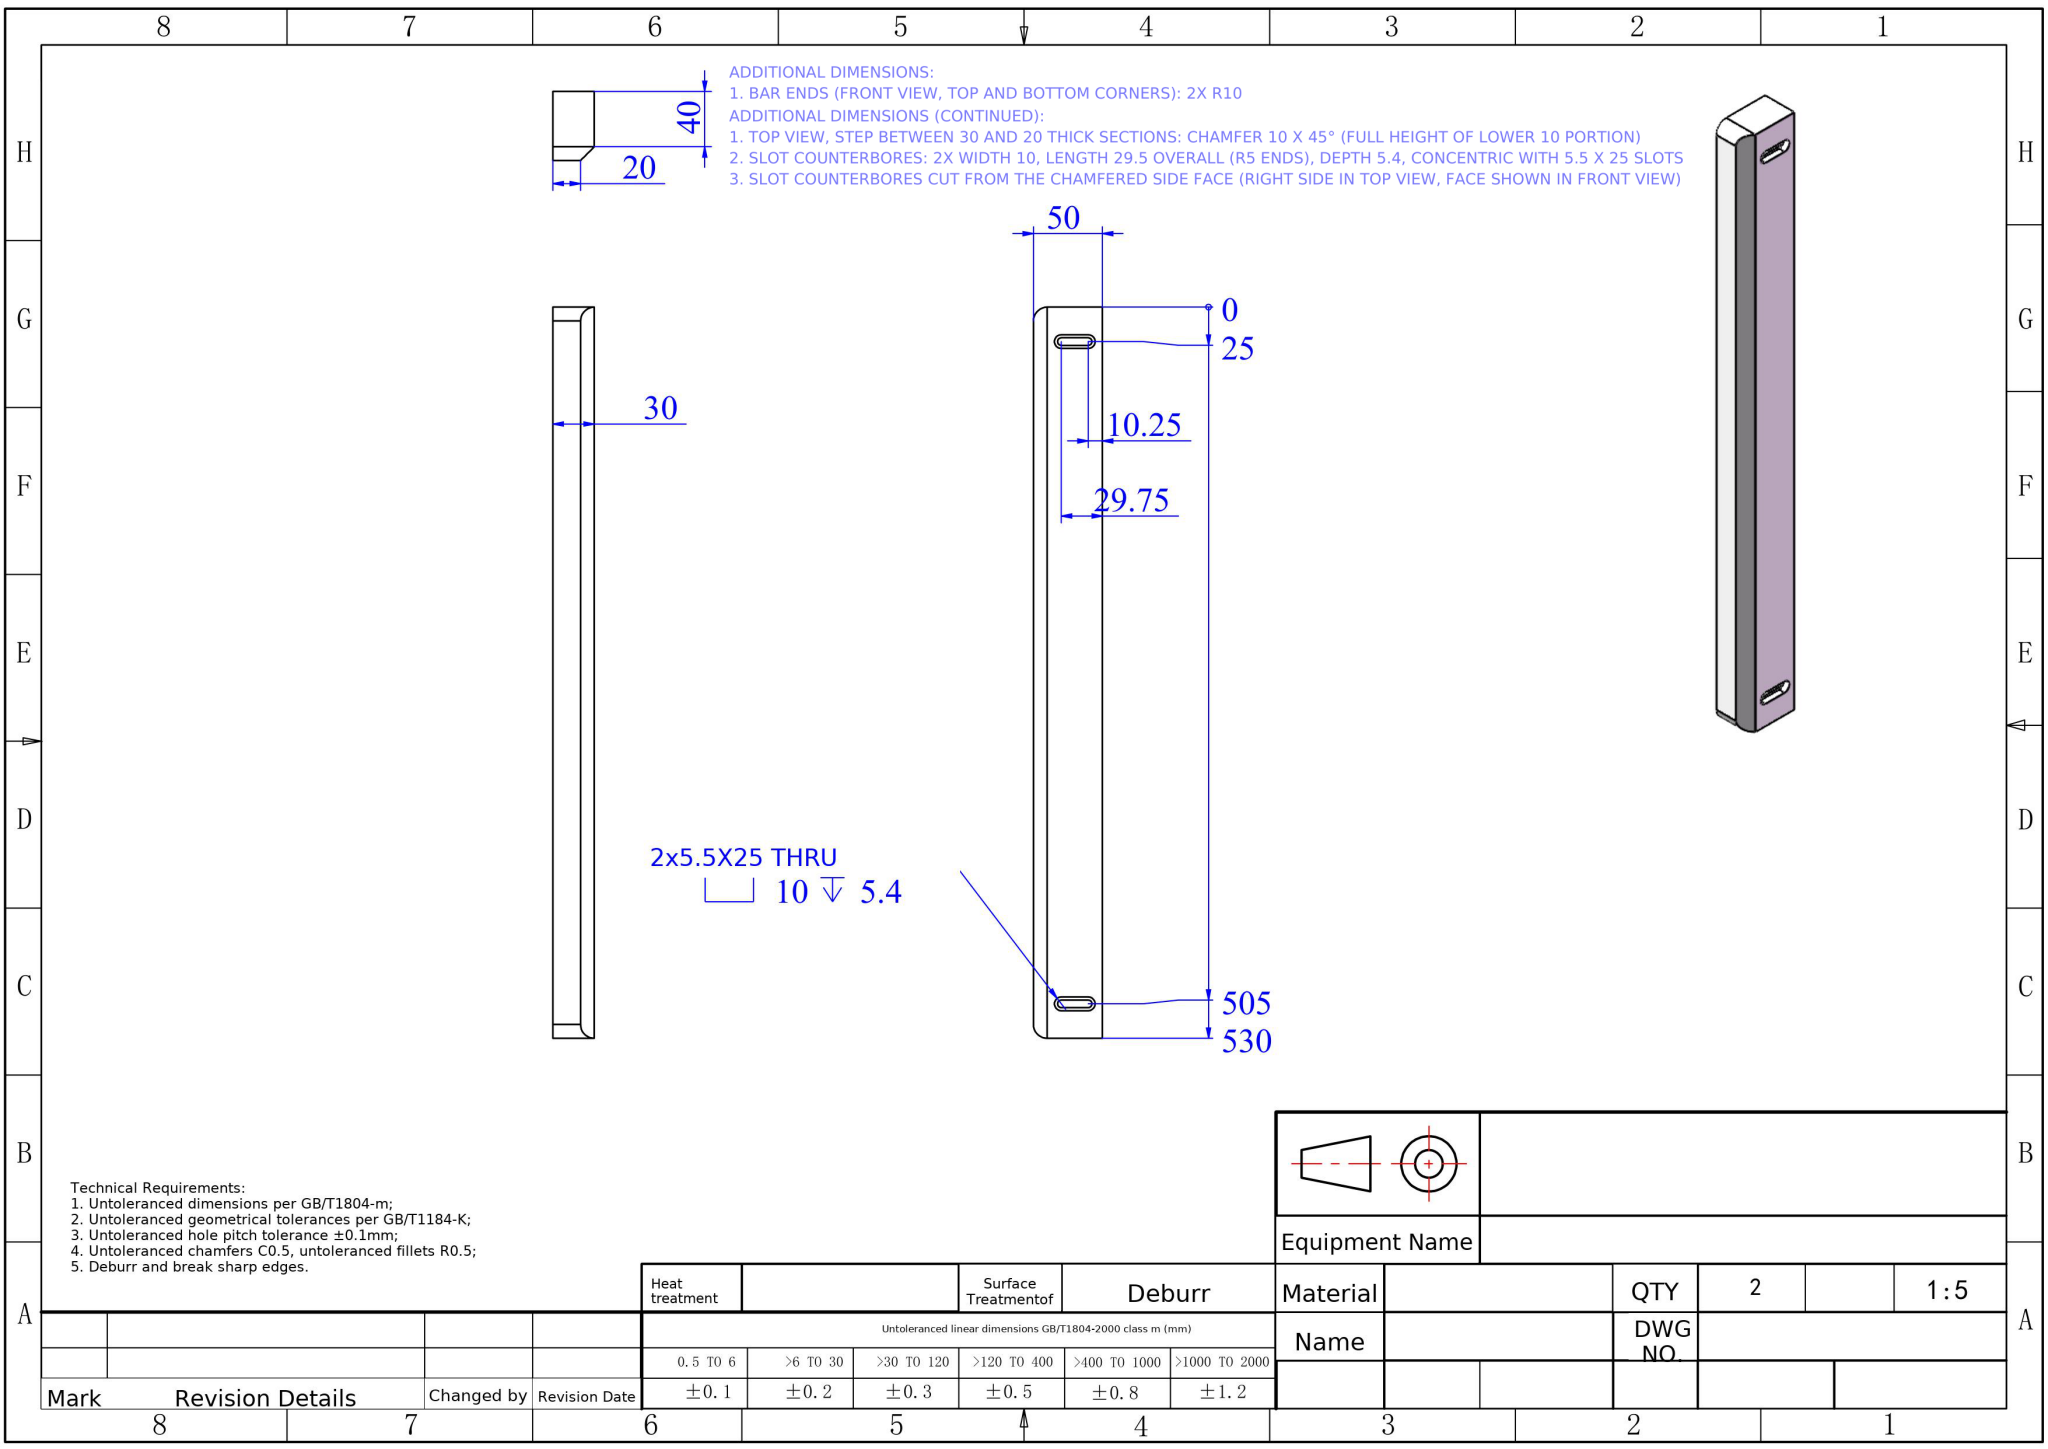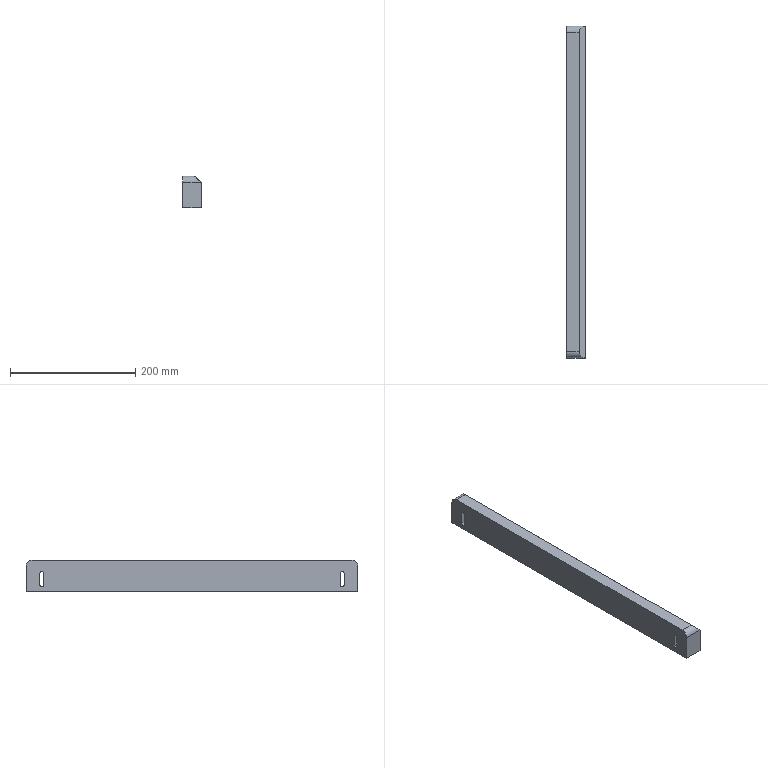Part | NX | mm | 1 solid | 31 faces | box 30 x 530 x 50 mm | volume 758146 mm3 | plane 17 | cylinder 14 | commonest cylinder face diameters 10 x6 5.5 x6 20 x2
STEP:
#1=CARTESIAN_POINT('',(9.6,-240.,5.25));
#2=VERTEX_POINT('',#1);
#3=CARTESIAN_POINT('',(9.6,-235.,10.25));
#4=VERTEX_POINT('',#3);
#5=CARTESIAN_POINT('',(9.6,-240.,10.25));
#6=DIRECTION('',(1.,0.,0.));
#7=DIRECTION('',(0.,0.,-1.));
#8=AXIS2_PLACEMENT_3D('',#5,#6,#7);
#9=CIRCLE('',#8,5.);
#10=EDGE_CURVE('',#2,#4,#9,.T.);
#11=ORIENTED_EDGE('',*,*,#10,.F.);
#12=CARTESIAN_POINT('',(15.,-240.,5.25));
#13=VERTEX_POINT('',#12);
#14=CARTESIAN_POINT('',(15.,-240.,5.25));
#15=DIRECTION('',(1.,0.,0.));
#16=VECTOR('',#15,1000.);
#17=LINE('',#14,#16);
#18=EDGE_CURVE('',#2,#13,#17,.T.);
#19=ORIENTED_EDGE('',*,*,#18,.T.);
#20=CARTESIAN_POINT('',(15.,-235.,10.25));
#21=VERTEX_POINT('',#20);
#22=CARTESIAN_POINT('',(15.,-240.,10.25));
#23=DIRECTION('',(1.,0.,0.));
#24=DIRECTION('',(0.,0.,-1.));
#25=AXIS2_PLACEMENT_3D('',#22,#23,#24);
#26=CIRCLE('',#25,5.);
#27=EDGE_CURVE('',#13,#21,#26,.T.);
#28=ORIENTED_EDGE('',*,*,#27,.T.);
#29=CARTESIAN_POINT('',(9.6,-235.,10.25));
#30=DIRECTION('',(-1.,-0.,0.));
#31=VECTOR('',#30,1000.);
#32=LINE('',#29,#31);
#33=EDGE_CURVE('',#21,#4,#32,.T.);
#34=ORIENTED_EDGE('',*,*,#33,.T.);
#35=EDGE_LOOP('',(#11,#19,#28,#34));
#36=FACE_OUTER_BOUND('',#35,.T.);
#37=CARTESIAN_POINT('',(15.,-240.,10.25));
#38=DIRECTION('',(1.,0.,0.));
#39=DIRECTION('',(0.,0.,-1.));
#40=AXIS2_PLACEMENT_3D('',#37,#38,#39);
#41=CYLINDRICAL_SURFACE('',#40,5.);
#42=ADVANCED_FACE('',(#36),#41,.F.);
#43=CARTESIAN_POINT('',(-15.,-240.,7.5));
#44=VERTEX_POINT('',#43);
#45=CARTESIAN_POINT('',(-15.,-237.25,10.25));
#46=VERTEX_POINT('',#45);
#47=CARTESIAN_POINT('',(-15.,-240.,10.25));
#48=DIRECTION('',(1.,0.,0.));
#49=DIRECTION('',(0.,0.,-1.));
#50=AXIS2_PLACEMENT_3D('',#47,#48,#49);
#51=CIRCLE('',#50,2.75);
#52=EDGE_CURVE('',#44,#46,#51,.T.);
#53=ORIENTED_EDGE('',*,*,#52,.F.);
#54=CARTESIAN_POINT('',(9.6,-240.,7.5));
#55=VERTEX_POINT('',#54);
#56=CARTESIAN_POINT('',(15.,-240.,7.5));
#57=DIRECTION('',(1.,0.,0.));
#58=VECTOR('',#57,1000.);
#59=LINE('',#56,#58);
#60=EDGE_CURVE('',#44,#55,#59,.T.);
#61=ORIENTED_EDGE('',*,*,#60,.T.);
#62=CARTESIAN_POINT('',(9.6,-237.25,10.25));
#63=VERTEX_POINT('',#62);
#64=CARTESIAN_POINT('',(9.6,-240.,10.25));
#65=DIRECTION('',(1.,0.,0.));
#66=DIRECTION('',(0.,0.,-1.));
#67=AXIS2_PLACEMENT_3D('',#64,#65,#66);
#68=CIRCLE('',#67,2.75);
#69=EDGE_CURVE('',#55,#63,#68,.T.);
#70=ORIENTED_EDGE('',*,*,#69,.T.);
#71=CARTESIAN_POINT('',(-15.,-237.25,10.25));
#72=DIRECTION('',(-1.,-0.,0.));
#73=VECTOR('',#72,1000.);
#74=LINE('',#71,#73);
#75=EDGE_CURVE('',#63,#46,#74,.T.);
#76=ORIENTED_EDGE('',*,*,#75,.T.);
#77=EDGE_LOOP('',(#53,#61,#70,#76));
#78=FACE_OUTER_BOUND('',#77,.T.);
#79=CARTESIAN_POINT('',(15.,-240.,10.25));
#80=DIRECTION('',(1.,0.,0.));
#81=DIRECTION('',(0.,0.,-1.));
#82=AXIS2_PLACEMENT_3D('',#79,#80,#81);
#83=CYLINDRICAL_SURFACE('',#82,2.75);
#84=ADVANCED_FACE('',(#78),#83,.F.);
#85=CARTESIAN_POINT('',(9.6,240.,5.25));
#86=VERTEX_POINT('',#85);
#87=CARTESIAN_POINT('',(9.6,245.,10.25));
#88=VERTEX_POINT('',#87);
#89=CARTESIAN_POINT('',(9.6,240.,10.25));
#90=DIRECTION('',(1.,0.,0.));
#91=DIRECTION('',(0.,0.,-1.));
#92=AXIS2_PLACEMENT_3D('',#89,#90,#91);
#93=CIRCLE('',#92,5.);
#94=EDGE_CURVE('',#86,#88,#93,.T.);
#95=ORIENTED_EDGE('',*,*,#94,.F.);
#96=CARTESIAN_POINT('',(15.,240.,5.25));
#97=VERTEX_POINT('',#96);
#98=CARTESIAN_POINT('',(15.,240.,5.25));
#99=DIRECTION('',(1.,0.,0.));
#100=VECTOR('',#99,1000.);
#101=LINE('',#98,#100);
#102=EDGE_CURVE('',#86,#97,#101,.T.);
#103=ORIENTED_EDGE('',*,*,#102,.T.);
#104=CARTESIAN_POINT('',(15.,245.,10.25));
#105=VERTEX_POINT('',#104);
#106=CARTESIAN_POINT('',(15.,240.,10.25));
#107=DIRECTION('',(1.,0.,0.));
#108=DIRECTION('',(0.,0.,-1.));
#109=AXIS2_PLACEMENT_3D('',#106,#107,#108);
#110=CIRCLE('',#109,5.);
#111=EDGE_CURVE('',#97,#105,#110,.T.);
#112=ORIENTED_EDGE('',*,*,#111,.T.);
#113=CARTESIAN_POINT('',(9.6,245.,10.25));
#114=DIRECTION('',(-1.,-0.,0.));
#115=VECTOR('',#114,1000.);
#116=LINE('',#113,#115);
#117=EDGE_CURVE('',#105,#88,#116,.T.);
#118=ORIENTED_EDGE('',*,*,#117,.T.);
#119=EDGE_LOOP('',(#95,#103,#112,#118));
#120=FACE_OUTER_BOUND('',#119,.T.);
#121=CARTESIAN_POINT('',(15.,240.,10.25));
#122=DIRECTION('',(1.,0.,0.));
#123=DIRECTION('',(0.,0.,-1.));
#124=AXIS2_PLACEMENT_3D('',#121,#122,#123);
#125=CYLINDRICAL_SURFACE('',#124,5.);
#126=ADVANCED_FACE('',(#120),#125,.F.);
#127=CARTESIAN_POINT('',(-15.,240.,7.5));
#128=VERTEX_POINT('',#127);
#129=CARTESIAN_POINT('',(-15.,242.75,10.25));
#130=VERTEX_POINT('',#129);
#131=CARTESIAN_POINT('',(-15.,240.,10.25));
#132=DIRECTION('',(1.,0.,0.));
#133=DIRECTION('',(0.,0.,-1.));
#134=AXIS2_PLACEMENT_3D('',#131,#132,#133);
#135=CIRCLE('',#134,2.75);
#136=EDGE_CURVE('',#128,#130,#135,.T.);
#137=ORIENTED_EDGE('',*,*,#136,.F.);
#138=CARTESIAN_POINT('',(9.6,240.,7.5));
#139=VERTEX_POINT('',#138);
#140=CARTESIAN_POINT('',(15.,240.,7.5));
#141=DIRECTION('',(1.,0.,0.));
#142=VECTOR('',#141,1000.);
#143=LINE('',#140,#142);
#144=EDGE_CURVE('',#128,#139,#143,.T.);
#145=ORIENTED_EDGE('',*,*,#144,.T.);
#146=CARTESIAN_POINT('',(9.6,242.75,10.25));
#147=VERTEX_POINT('',#146);
#148=CARTESIAN_POINT('',(9.6,240.,10.25));
#149=DIRECTION('',(1.,0.,0.));
#150=DIRECTION('',(0.,0.,-1.));
#151=AXIS2_PLACEMENT_3D('',#148,#149,#150);
#152=CIRCLE('',#151,2.75);
#153=EDGE_CURVE('',#139,#147,#152,.T.);
#154=ORIENTED_EDGE('',*,*,#153,.T.);
#155=CARTESIAN_POINT('',(-15.,242.75,10.25));
#156=DIRECTION('',(-1.,-0.,0.));
#157=VECTOR('',#156,1000.);
#158=LINE('',#155,#157);
#159=EDGE_CURVE('',#147,#130,#158,.T.);
#160=ORIENTED_EDGE('',*,*,#159,.T.);
#161=EDGE_LOOP('',(#137,#145,#154,#160));
#162=FACE_OUTER_BOUND('',#161,.T.);
#163=CARTESIAN_POINT('',(15.,240.,10.25));
#164=DIRECTION('',(1.,0.,0.));
#165=DIRECTION('',(0.,0.,-1.));
#166=AXIS2_PLACEMENT_3D('',#163,#164,#165);
#167=CYLINDRICAL_SURFACE('',#166,2.75);
#168=ADVANCED_FACE('',(#162),#167,.F.);
#169=CARTESIAN_POINT('',(15.,-245.,10.25));
#170=VERTEX_POINT('',#169);
#171=CARTESIAN_POINT('',(15.,-240.,10.25));
#172=DIRECTION('',(1.,0.,0.));
#173=DIRECTION('',(0.,0.,-1.));
#174=AXIS2_PLACEMENT_3D('',#171,#172,#173);
#175=CIRCLE('',#174,5.);
#176=EDGE_CURVE('',#170,#13,#175,.T.);
#177=ORIENTED_EDGE('',*,*,#176,.F.);
#178=CARTESIAN_POINT('',(15.,-245.,29.75));
#179=VERTEX_POINT('',#178);
#180=CARTESIAN_POINT('',(15.,-245.,10.25));
#181=DIRECTION('',(0.,0.,1.));
#182=VECTOR('',#181,1000.);
#183=LINE('',#180,#182);
#184=EDGE_CURVE('',#170,#179,#183,.T.);
#185=ORIENTED_EDGE('',*,*,#184,.T.);
#186=CARTESIAN_POINT('',(15.,-235.,29.75));
#187=VERTEX_POINT('',#186);
#188=CARTESIAN_POINT('',(15.,-240.,29.75));
#189=DIRECTION('',(1.,0.,0.));
#190=DIRECTION('',(0.,0.,-1.));
#191=AXIS2_PLACEMENT_3D('',#188,#189,#190);
#192=CIRCLE('',#191,5.);
#193=EDGE_CURVE('',#187,#179,#192,.T.);
#194=ORIENTED_EDGE('',*,*,#193,.F.);
#195=CARTESIAN_POINT('',(15.,-235.,10.25));
#196=DIRECTION('',(0.,0.,1.));
#197=VECTOR('',#196,1000.);
#198=LINE('',#195,#197);
#199=EDGE_CURVE('',#21,#187,#198,.T.);
#200=ORIENTED_EDGE('',*,*,#199,.F.);
#201=ORIENTED_EDGE('',*,*,#27,.F.);
#202=EDGE_LOOP('',(#177,#185,#194,#200,#201));
#203=FACE_BOUND('',#202,.T.);
#204=CARTESIAN_POINT('',(15.,265.,40.));
#205=VERTEX_POINT('',#204);
#206=CARTESIAN_POINT('',(15.,265.,0.));
#207=VERTEX_POINT('',#206);
#208=CARTESIAN_POINT('',(15.,265.,50.));
#209=DIRECTION('',(0.,0.,-1.));
#210=VECTOR('',#209,1000.);
#211=LINE('',#208,#210);
#212=EDGE_CURVE('',#205,#207,#211,.T.);
#213=ORIENTED_EDGE('',*,*,#212,.F.);
#214=CARTESIAN_POINT('',(15.,-265.,40.));
#215=VERTEX_POINT('',#214);
#216=CARTESIAN_POINT('',(15.,-265.,40.));
#217=DIRECTION('',(0.,-1.,0.));
#218=VECTOR('',#217,1000.);
#219=LINE('',#216,#218);
#220=EDGE_CURVE('',#205,#215,#219,.T.);
#221=ORIENTED_EDGE('',*,*,#220,.T.);
#222=CARTESIAN_POINT('',(15.,-265.,0.));
#223=VERTEX_POINT('',#222);
#224=CARTESIAN_POINT('',(15.,-265.,50.));
#225=DIRECTION('',(0.,0.,-1.));
#226=VECTOR('',#225,1000.);
#227=LINE('',#224,#226);
#228=EDGE_CURVE('',#215,#223,#227,.T.);
#229=ORIENTED_EDGE('',*,*,#228,.T.);
#230=CARTESIAN_POINT('',(15.,-265.,0.));
#231=DIRECTION('',(0.,1.,0.));
#232=VECTOR('',#231,1000.);
#233=LINE('',#230,#232);
#234=EDGE_CURVE('',#223,#207,#233,.T.);
#235=ORIENTED_EDGE('',*,*,#234,.T.);
#236=EDGE_LOOP('',(#213,#221,#229,#235));
#237=FACE_OUTER_BOUND('',#236,.T.);
#238=CARTESIAN_POINT('',(15.,245.,29.75));
#239=VERTEX_POINT('',#238);
#240=CARTESIAN_POINT('',(15.,245.,10.25));
#241=DIRECTION('',(0.,0.,1.));
#242=VECTOR('',#241,1000.);
#243=LINE('',#240,#242);
#244=EDGE_CURVE('',#105,#239,#243,.T.);
#245=ORIENTED_EDGE('',*,*,#244,.F.);
#246=ORIENTED_EDGE('',*,*,#111,.F.);
#247=CARTESIAN_POINT('',(15.,235.,10.25));
#248=VERTEX_POINT('',#247);
#249=CARTESIAN_POINT('',(15.,240.,10.25));
#250=DIRECTION('',(1.,0.,0.));
#251=DIRECTION('',(0.,0.,-1.));
#252=AXIS2_PLACEMENT_3D('',#249,#250,#251);
#253=CIRCLE('',#252,5.);
#254=EDGE_CURVE('',#248,#97,#253,.T.);
#255=ORIENTED_EDGE('',*,*,#254,.F.);
#256=CARTESIAN_POINT('',(15.,235.,29.75));
#257=VERTEX_POINT('',#256);
#258=CARTESIAN_POINT('',(15.,235.,10.25));
#259=DIRECTION('',(0.,0.,1.));
#260=VECTOR('',#259,1000.);
#261=LINE('',#258,#260);
#262=EDGE_CURVE('',#248,#257,#261,.T.);
#263=ORIENTED_EDGE('',*,*,#262,.T.);
#264=CARTESIAN_POINT('',(15.,240.,29.75));
#265=DIRECTION('',(1.,0.,0.));
#266=DIRECTION('',(0.,0.,-1.));
#267=AXIS2_PLACEMENT_3D('',#264,#265,#266);
#268=CIRCLE('',#267,5.);
#269=EDGE_CURVE('',#239,#257,#268,.T.);
#270=ORIENTED_EDGE('',*,*,#269,.F.);
#271=EDGE_LOOP('',(#245,#246,#255,#263,#270));
#272=FACE_BOUND('',#271,.T.);
#273=CARTESIAN_POINT('',(15.,-265.,50.));
#274=DIRECTION('',(-1.,0.,0.));
#275=DIRECTION('',(0.,0.,1.));
#276=AXIS2_PLACEMENT_3D('',#273,#274,#275);
#277=PLANE('',#276);
#278=ADVANCED_FACE('',(#203,#237,#272),#277,.F.);
#279=CARTESIAN_POINT('',(-15.,265.,40.));
#280=VERTEX_POINT('',#279);
#281=CARTESIAN_POINT('',(-15.,265.,0.));
#282=VERTEX_POINT('',#281);
#283=CARTESIAN_POINT('',(-15.,265.,50.));
#284=DIRECTION('',(0.,0.,-1.));
#285=VECTOR('',#284,1000.);
#286=LINE('',#283,#285);
#287=EDGE_CURVE('',#280,#282,#286,.T.);
#288=ORIENTED_EDGE('',*,*,#287,.F.);
#289=CARTESIAN_POINT('',(-15.,265.,40.));
#290=DIRECTION('',(1.,0.,0.));
#291=VECTOR('',#290,1000.);
#292=LINE('',#289,#291);
#293=EDGE_CURVE('',#280,#205,#292,.T.);
#294=ORIENTED_EDGE('',*,*,#293,.T.);
#295=ORIENTED_EDGE('',*,*,#212,.T.);
#296=CARTESIAN_POINT('',(-15.,265.,0.));
#297=DIRECTION('',(-1.,0.,0.));
#298=VECTOR('',#297,1000.);
#299=LINE('',#296,#298);
#300=EDGE_CURVE('',#207,#282,#299,.T.);
#301=ORIENTED_EDGE('',*,*,#300,.T.);
#302=EDGE_LOOP('',(#288,#294,#295,#301));
#303=FACE_OUTER_BOUND('',#302,.T.);
#304=CARTESIAN_POINT('',(-15.,265.,50.));
#305=DIRECTION('',(0.,-1.,0.));
#306=DIRECTION('',(0.,0.,-1.));
#307=AXIS2_PLACEMENT_3D('',#304,#305,#306);
#308=PLANE('',#307);
#309=ADVANCED_FACE('',(#303),#308,.F.);
#310=CARTESIAN_POINT('',(-15.,-242.75,10.25));
#311=VERTEX_POINT('',#310);
#312=CARTESIAN_POINT('',(-15.,-242.75,29.75));
#313=VERTEX_POINT('',#312);
#314=CARTESIAN_POINT('',(-15.,-242.75,10.25));
#315=DIRECTION('',(0.,0.,1.));
#316=VECTOR('',#315,1000.);
#317=LINE('',#314,#316);
#318=EDGE_CURVE('',#311,#313,#317,.T.);
#319=ORIENTED_EDGE('',*,*,#318,.F.);
#320=CARTESIAN_POINT('',(-15.,-240.,10.25));
#321=DIRECTION('',(1.,0.,0.));
#322=DIRECTION('',(0.,0.,-1.));
#323=AXIS2_PLACEMENT_3D('',#320,#321,#322);
#324=CIRCLE('',#323,2.75);
#325=EDGE_CURVE('',#311,#44,#324,.T.);
#326=ORIENTED_EDGE('',*,*,#325,.T.);
#327=ORIENTED_EDGE('',*,*,#52,.T.);
#328=CARTESIAN_POINT('',(-15.,-237.25,29.75));
#329=VERTEX_POINT('',#328);
#330=CARTESIAN_POINT('',(-15.,-237.25,10.25));
#331=DIRECTION('',(0.,0.,1.));
#332=VECTOR('',#331,1000.);
#333=LINE('',#330,#332);
#334=EDGE_CURVE('',#46,#329,#333,.T.);
#335=ORIENTED_EDGE('',*,*,#334,.T.);
#336=CARTESIAN_POINT('',(-15.,-240.,29.75));
#337=DIRECTION('',(1.,0.,0.));
#338=DIRECTION('',(0.,0.,-1.));
#339=AXIS2_PLACEMENT_3D('',#336,#337,#338);
#340=CIRCLE('',#339,2.75);
#341=EDGE_CURVE('',#329,#313,#340,.T.);
#342=ORIENTED_EDGE('',*,*,#341,.T.);
#343=EDGE_LOOP('',(#319,#326,#327,#335,#342));
#344=FACE_BOUND('',#343,.T.);
#345=CARTESIAN_POINT('',(-15.,242.75,29.75));
#346=VERTEX_POINT('',#345);
#347=CARTESIAN_POINT('',(-15.,242.75,10.25));
#348=DIRECTION('',(0.,0.,1.));
#349=VECTOR('',#348,1000.);
#350=LINE('',#347,#349);
#351=EDGE_CURVE('',#130,#346,#350,.T.);
#352=ORIENTED_EDGE('',*,*,#351,.T.);
#353=CARTESIAN_POINT('',(-15.,237.25,29.75));
#354=VERTEX_POINT('',#353);
#355=CARTESIAN_POINT('',(-15.,240.,29.75));
#356=DIRECTION('',(1.,0.,0.));
#357=DIRECTION('',(0.,0.,-1.));
#358=AXIS2_PLACEMENT_3D('',#355,#356,#357);
#359=CIRCLE('',#358,2.75);
#360=EDGE_CURVE('',#346,#354,#359,.T.);
#361=ORIENTED_EDGE('',*,*,#360,.T.);
#362=CARTESIAN_POINT('',(-15.,237.25,10.25));
#363=VERTEX_POINT('',#362);
#364=CARTESIAN_POINT('',(-15.,237.25,10.25));
#365=DIRECTION('',(0.,0.,1.));
#366=VECTOR('',#365,1000.);
#367=LINE('',#364,#366);
#368=EDGE_CURVE('',#363,#354,#367,.T.);
#369=ORIENTED_EDGE('',*,*,#368,.F.);
#370=CARTESIAN_POINT('',(-15.,240.,10.25));
#371=DIRECTION('',(1.,0.,0.));
#372=DIRECTION('',(0.,0.,-1.));
#373=AXIS2_PLACEMENT_3D('',#370,#371,#372);
#374=CIRCLE('',#373,2.75);
#375=EDGE_CURVE('',#363,#128,#374,.T.);
#376=ORIENTED_EDGE('',*,*,#375,.T.);
#377=ORIENTED_EDGE('',*,*,#136,.T.);
#378=EDGE_LOOP('',(#352,#361,#369,#376,#377));
#379=FACE_BOUND('',#378,.T.);
#380=CARTESIAN_POINT('',(-15.,-265.,40.));
#381=VERTEX_POINT('',#380);
#382=CARTESIAN_POINT('',(-15.,-265.,0.));
#383=VERTEX_POINT('',#382);
#384=CARTESIAN_POINT('',(-15.,-265.,50.));
#385=DIRECTION('',(0.,0.,-1.));
#386=VECTOR('',#385,1000.);
#387=LINE('',#384,#386);
#388=EDGE_CURVE('',#381,#383,#387,.T.);
#389=ORIENTED_EDGE('',*,*,#388,.F.);
#390=CARTESIAN_POINT('',(-15.,-255.,50.));
#391=VERTEX_POINT('',#390);
#392=CARTESIAN_POINT('',(-15.,-255.,40.));
#393=DIRECTION('',(-1.,0.,0.));
#394=DIRECTION('',(0.,0.,-1.));
#395=AXIS2_PLACEMENT_3D('',#392,#393,#394);
#396=CIRCLE('',#395,10.);
#397=EDGE_CURVE('',#381,#391,#396,.T.);
#398=ORIENTED_EDGE('',*,*,#397,.T.);
#399=CARTESIAN_POINT('',(-15.,255.,50.));
#400=VERTEX_POINT('',#399);
#401=CARTESIAN_POINT('',(-15.,-265.,50.));
#402=DIRECTION('',(0.,-1.,0.));
#403=VECTOR('',#402,1000.);
#404=LINE('',#401,#403);
#405=EDGE_CURVE('',#400,#391,#404,.T.);
#406=ORIENTED_EDGE('',*,*,#405,.F.);
#407=CARTESIAN_POINT('',(-15.,255.,40.));
#408=DIRECTION('',(-1.,0.,0.));
#409=DIRECTION('',(0.,0.,-1.));
#410=AXIS2_PLACEMENT_3D('',#407,#408,#409);
#411=CIRCLE('',#410,10.);
#412=EDGE_CURVE('',#400,#280,#411,.T.);
#413=ORIENTED_EDGE('',*,*,#412,.T.);
#414=ORIENTED_EDGE('',*,*,#287,.T.);
#415=CARTESIAN_POINT('',(-15.,-265.,0.));
#416=DIRECTION('',(0.,-1.,0.));
#417=VECTOR('',#416,1000.);
#418=LINE('',#415,#417);
#419=EDGE_CURVE('',#282,#383,#418,.T.);
#420=ORIENTED_EDGE('',*,*,#419,.T.);
#421=EDGE_LOOP('',(#389,#398,#406,#413,#414,#420));
#422=FACE_OUTER_BOUND('',#421,.T.);
#423=CARTESIAN_POINT('',(-15.,-265.,50.));
#424=DIRECTION('',(1.,0.,0.));
#425=DIRECTION('',(0.,0.,-1.));
#426=AXIS2_PLACEMENT_3D('',#423,#424,#425);
#427=PLANE('',#426);
#428=ADVANCED_FACE('',(#344,#379,#422),#427,.F.);
#429=ORIENTED_EDGE('',*,*,#228,.F.);
#430=CARTESIAN_POINT('',(-15.,-265.,40.));
#431=DIRECTION('',(-1.,0.,0.));
#432=VECTOR('',#431,1000.);
#433=LINE('',#430,#432);
#434=EDGE_CURVE('',#215,#381,#433,.T.);
#435=ORIENTED_EDGE('',*,*,#434,.T.);
#436=ORIENTED_EDGE('',*,*,#388,.T.);
#437=CARTESIAN_POINT('',(-15.,-265.,0.));
#438=DIRECTION('',(1.,0.,0.));
#439=VECTOR('',#438,1000.);
#440=LINE('',#437,#439);
#441=EDGE_CURVE('',#383,#223,#440,.T.);
#442=ORIENTED_EDGE('',*,*,#441,.T.);
#443=EDGE_LOOP('',(#429,#435,#436,#442));
#444=FACE_OUTER_BOUND('',#443,.T.);
#445=CARTESIAN_POINT('',(-15.,-265.,50.));
#446=DIRECTION('',(0.,1.,0.));
#447=DIRECTION('',(0.,0.,1.));
#448=AXIS2_PLACEMENT_3D('',#445,#446,#447);
#449=PLANE('',#448);
#450=ADVANCED_FACE('',(#444),#449,.F.);
#451=ORIENTED_EDGE('',*,*,#405,.T.);
#452=CARTESIAN_POINT('',(5.,-255.,50.));
#453=VERTEX_POINT('',#452);
#454=CARTESIAN_POINT('',(0.,-255.,50.));
#455=DIRECTION('',(1.,0.,0.));
#456=VECTOR('',#455,1000.);
#457=LINE('',#454,#456);
#458=EDGE_CURVE('',#391,#453,#457,.T.);
#459=ORIENTED_EDGE('',*,*,#458,.T.);
#460=CARTESIAN_POINT('',(5.,255.,50.));
#461=VERTEX_POINT('',#460);
#462=CARTESIAN_POINT('',(5.,0.,50.));
#463=DIRECTION('',(0.,1.,0.));
#464=VECTOR('',#463,1000.);
#465=LINE('',#462,#464);
#466=EDGE_CURVE('',#453,#461,#465,.T.);
#467=ORIENTED_EDGE('',*,*,#466,.T.);
#468=CARTESIAN_POINT('',(0.,255.,50.));
#469=DIRECTION('',(-1.,0.,0.));
#470=VECTOR('',#469,1000.);
#471=LINE('',#468,#470);
#472=EDGE_CURVE('',#461,#400,#471,.T.);
#473=ORIENTED_EDGE('',*,*,#472,.T.);
#474=EDGE_LOOP('',(#451,#459,#467,#473));
#475=FACE_OUTER_BOUND('',#474,.T.);
#476=CARTESIAN_POINT('',(0.,0.,50.));
#477=DIRECTION('',(0.,0.,-1.));
#478=DIRECTION('',(-1.,0.,0.));
#479=AXIS2_PLACEMENT_3D('',#476,#477,#478);
#480=PLANE('',#479);
#481=ADVANCED_FACE('',(#475),#480,.F.);
#482=ORIENTED_EDGE('',*,*,#234,.F.);
#483=ORIENTED_EDGE('',*,*,#441,.F.);
#484=ORIENTED_EDGE('',*,*,#419,.F.);
#485=ORIENTED_EDGE('',*,*,#300,.F.);
#486=EDGE_LOOP('',(#482,#483,#484,#485));
#487=FACE_OUTER_BOUND('',#486,.T.);
#488=CARTESIAN_POINT('',(0.,0.,0.));
#489=DIRECTION('',(0.,0.,-1.));
#490=DIRECTION('',(-1.,0.,0.));
#491=AXIS2_PLACEMENT_3D('',#488,#489,#490);
#492=PLANE('',#491);
#493=ADVANCED_FACE('',(#487),#492,.T.);
#494=ORIENTED_EDGE('',*,*,#466,.F.);
#495=CARTESIAN_POINT('',(5.,-255.,50.));
#496=CARTESIAN_POINT('',(5.,-260.858,50.));
#497=CARTESIAN_POINT('',(9.142,-265.,45.858));
#498=CARTESIAN_POINT('',(15.,-265.,40.));
#499=(BOUNDED_CURVE()B_SPLINE_CURVE(3,(#495,#496,#497,#498),.UNSPECIFIED.,.F.,.F.)B_SPLINE_CURVE_WITH_KNOTS((4,4),(3.142,4.712),.UNSPECIFIED.)CURVE()GEOMETRIC_REPRESENTATION_ITEM()RATIONAL_B_SPLINE_CURVE((1.,0.8047,0.8047,1.))REPRESENTATION_ITEM(''));
#500=EDGE_CURVE('',#453,#215,#499,.T.);
#501=ORIENTED_EDGE('',*,*,#500,.T.);
#502=ORIENTED_EDGE('',*,*,#220,.F.);
#503=CARTESIAN_POINT('',(15.,265.,40.));
#504=CARTESIAN_POINT('',(9.142,265.,45.858));
#505=CARTESIAN_POINT('',(5.,260.858,50.));
#506=CARTESIAN_POINT('',(5.,255.,50.));
#507=(BOUNDED_CURVE()B_SPLINE_CURVE(3,(#503,#504,#505,#506),.UNSPECIFIED.,.F.,.T.)B_SPLINE_CURVE_WITH_KNOTS((4,4),(4.712,6.283),.UNSPECIFIED.)CURVE()GEOMETRIC_REPRESENTATION_ITEM()RATIONAL_B_SPLINE_CURVE((1.,0.8047,0.8047,1.))REPRESENTATION_ITEM(''));
#508=EDGE_CURVE('',#205,#461,#507,.T.);
#509=ORIENTED_EDGE('',*,*,#508,.T.);
#510=EDGE_LOOP('',(#494,#501,#502,#509));
#511=FACE_OUTER_BOUND('',#510,.T.);
#512=CARTESIAN_POINT('',(5.,0.,50.));
#513=DIRECTION('',(-0.7071,0.,-0.7071));
#514=DIRECTION('',(0.,1.,0.));
#515=AXIS2_PLACEMENT_3D('',#512,#513,#514);
#516=PLANE('',#515);
#517=ADVANCED_FACE('',(#511),#516,.F.);
#518=ORIENTED_EDGE('',*,*,#397,.F.);
#519=ORIENTED_EDGE('',*,*,#434,.F.);
#520=ORIENTED_EDGE('',*,*,#500,.F.);
#521=ORIENTED_EDGE('',*,*,#458,.F.);
#522=EDGE_LOOP('',(#518,#519,#520,#521));
#523=FACE_OUTER_BOUND('',#522,.T.);
#524=CARTESIAN_POINT('',(0.,-255.,40.));
#525=DIRECTION('',(1.,0.,0.));
#526=DIRECTION('',(0.,0.,-1.));
#527=AXIS2_PLACEMENT_3D('',#524,#525,#526);
#528=CYLINDRICAL_SURFACE('',#527,10.);
#529=ADVANCED_FACE('',(#523),#528,.T.);
#530=ORIENTED_EDGE('',*,*,#508,.F.);
#531=ORIENTED_EDGE('',*,*,#293,.F.);
#532=ORIENTED_EDGE('',*,*,#412,.F.);
#533=ORIENTED_EDGE('',*,*,#472,.F.);
#534=EDGE_LOOP('',(#530,#531,#532,#533));
#535=FACE_OUTER_BOUND('',#534,.T.);
#536=CARTESIAN_POINT('',(0.,255.,40.));
#537=DIRECTION('',(-1.,0.,0.));
#538=DIRECTION('',(0.,0.,1.));
#539=AXIS2_PLACEMENT_3D('',#536,#537,#538);
#540=CYLINDRICAL_SURFACE('',#539,10.);
#541=ADVANCED_FACE('',(#535),#540,.T.);
#542=ORIENTED_EDGE('',*,*,#360,.F.);
#543=CARTESIAN_POINT('',(9.6,242.75,29.75));
#544=VERTEX_POINT('',#543);
#545=CARTESIAN_POINT('',(-15.,242.75,29.75));
#546=DIRECTION('',(-1.,-0.,0.));
#547=VECTOR('',#546,1000.);
#548=LINE('',#545,#547);
#549=EDGE_CURVE('',#544,#346,#548,.T.);
#550=ORIENTED_EDGE('',*,*,#549,.F.);
#551=CARTESIAN_POINT('',(9.6,237.25,29.75));
#552=VERTEX_POINT('',#551);
#553=CARTESIAN_POINT('',(9.6,240.,29.75));
#554=DIRECTION('',(1.,0.,0.));
#555=DIRECTION('',(0.,0.,-1.));
#556=AXIS2_PLACEMENT_3D('',#553,#554,#555);
#557=CIRCLE('',#556,2.75);
#558=EDGE_CURVE('',#544,#552,#557,.T.);
#559=ORIENTED_EDGE('',*,*,#558,.T.);
#560=CARTESIAN_POINT('',(15.,237.25,29.75));
#561=DIRECTION('',(1.,0.,0.));
#562=VECTOR('',#561,1000.);
#563=LINE('',#560,#562);
#564=EDGE_CURVE('',#354,#552,#563,.T.);
#565=ORIENTED_EDGE('',*,*,#564,.F.);
#566=EDGE_LOOP('',(#542,#550,#559,#565));
#567=FACE_OUTER_BOUND('',#566,.T.);
#568=CARTESIAN_POINT('',(15.,240.,29.75));
#569=DIRECTION('',(1.,0.,0.));
#570=DIRECTION('',(0.,0.,-1.));
#571=AXIS2_PLACEMENT_3D('',#568,#569,#570);
#572=CYLINDRICAL_SURFACE('',#571,2.75);
#573=ADVANCED_FACE('',(#567),#572,.F.);
#574=CARTESIAN_POINT('',(9.6,235.,10.25));
#575=VERTEX_POINT('',#574);
#576=CARTESIAN_POINT('',(9.6,235.,29.75));
#577=VERTEX_POINT('',#576);
#578=CARTESIAN_POINT('',(9.6,235.,10.25));
#579=DIRECTION('',(0.,0.,1.));
#580=VECTOR('',#579,1000.);
#581=LINE('',#578,#580);
#582=EDGE_CURVE('',#575,#577,#581,.T.);
#583=ORIENTED_EDGE('',*,*,#582,.F.);
#584=CARTESIAN_POINT('',(9.6,240.,10.25));
#585=DIRECTION('',(1.,0.,0.));
#586=DIRECTION('',(0.,0.,-1.));
#587=AXIS2_PLACEMENT_3D('',#584,#585,#586);
#588=CIRCLE('',#587,5.);
#589=EDGE_CURVE('',#575,#86,#588,.T.);
#590=ORIENTED_EDGE('',*,*,#589,.T.);
#591=ORIENTED_EDGE('',*,*,#94,.T.);
#592=CARTESIAN_POINT('',(9.6,245.,29.75));
#593=VERTEX_POINT('',#592);
#594=CARTESIAN_POINT('',(9.6,245.,10.25));
#595=DIRECTION('',(0.,0.,1.));
#596=VECTOR('',#595,1000.);
#597=LINE('',#594,#596);
#598=EDGE_CURVE('',#88,#593,#597,.T.);
#599=ORIENTED_EDGE('',*,*,#598,.T.);
#600=CARTESIAN_POINT('',(9.6,240.,29.75));
#601=DIRECTION('',(1.,0.,0.));
#602=DIRECTION('',(0.,0.,-1.));
#603=AXIS2_PLACEMENT_3D('',#600,#601,#602);
#604=CIRCLE('',#603,5.);
#605=EDGE_CURVE('',#593,#577,#604,.T.);
#606=ORIENTED_EDGE('',*,*,#605,.T.);
#607=EDGE_LOOP('',(#583,#590,#591,#599,#606));
#608=FACE_OUTER_BOUND('',#607,.T.);
#609=ORIENTED_EDGE('',*,*,#558,.F.);
#610=CARTESIAN_POINT('',(9.6,242.75,10.25));
#611=DIRECTION('',(0.,0.,1.));
#612=VECTOR('',#611,1000.);
#613=LINE('',#610,#612);
#614=EDGE_CURVE('',#147,#544,#613,.T.);
#615=ORIENTED_EDGE('',*,*,#614,.F.);
#616=ORIENTED_EDGE('',*,*,#153,.F.);
#617=CARTESIAN_POINT('',(9.6,237.25,10.25));
#618=VERTEX_POINT('',#617);
#619=CARTESIAN_POINT('',(9.6,240.,10.25));
#620=DIRECTION('',(1.,0.,0.));
#621=DIRECTION('',(0.,0.,-1.));
#622=AXIS2_PLACEMENT_3D('',#619,#620,#621);
#623=CIRCLE('',#622,2.75);
#624=EDGE_CURVE('',#618,#139,#623,.T.);
#625=ORIENTED_EDGE('',*,*,#624,.F.);
#626=CARTESIAN_POINT('',(9.6,237.25,10.25));
#627=DIRECTION('',(0.,0.,1.));
#628=VECTOR('',#627,1000.);
#629=LINE('',#626,#628);
#630=EDGE_CURVE('',#618,#552,#629,.T.);
#631=ORIENTED_EDGE('',*,*,#630,.T.);
#632=EDGE_LOOP('',(#609,#615,#616,#625,#631));
#633=FACE_BOUND('',#632,.T.);
#634=CARTESIAN_POINT('',(9.6,242.75,29.75));
#635=DIRECTION('',(-1.,0.,0.));
#636=DIRECTION('',(0.,0.,1.));
#637=AXIS2_PLACEMENT_3D('',#634,#635,#636);
#638=PLANE('',#637);
#639=ADVANCED_FACE('',(#608,#633),#638,.F.);
#640=ORIENTED_EDGE('',*,*,#605,.F.);
#641=CARTESIAN_POINT('',(9.6,245.,29.75));
#642=DIRECTION('',(-1.,-0.,0.));
#643=VECTOR('',#642,1000.);
#644=LINE('',#641,#643);
#645=EDGE_CURVE('',#239,#593,#644,.T.);
#646=ORIENTED_EDGE('',*,*,#645,.F.);
#647=ORIENTED_EDGE('',*,*,#269,.T.);
#648=CARTESIAN_POINT('',(15.,235.,29.75));
#649=DIRECTION('',(1.,0.,0.));
#650=VECTOR('',#649,1000.);
#651=LINE('',#648,#650);
#652=EDGE_CURVE('',#577,#257,#651,.T.);
#653=ORIENTED_EDGE('',*,*,#652,.F.);
#654=EDGE_LOOP('',(#640,#646,#647,#653));
#655=FACE_OUTER_BOUND('',#654,.T.);
#656=CARTESIAN_POINT('',(15.,240.,29.75));
#657=DIRECTION('',(1.,0.,0.));
#658=DIRECTION('',(0.,0.,-1.));
#659=AXIS2_PLACEMENT_3D('',#656,#657,#658);
#660=CYLINDRICAL_SURFACE('',#659,5.);
#661=ADVANCED_FACE('',(#655),#660,.F.);
#662=ORIENTED_EDGE('',*,*,#144,.F.);
#663=ORIENTED_EDGE('',*,*,#375,.F.);
#664=CARTESIAN_POINT('',(15.,237.25,10.25));
#665=DIRECTION('',(-1.,0.,0.));
#666=VECTOR('',#665,1000.);
#667=LINE('',#664,#666);
#668=EDGE_CURVE('',#618,#363,#667,.T.);
#669=ORIENTED_EDGE('',*,*,#668,.F.);
#670=ORIENTED_EDGE('',*,*,#624,.T.);
#671=EDGE_LOOP('',(#662,#663,#669,#670));
#672=FACE_OUTER_BOUND('',#671,.T.);
#673=CARTESIAN_POINT('',(15.,240.,10.25));
#674=DIRECTION('',(1.,0.,0.));
#675=DIRECTION('',(0.,0.,-1.));
#676=AXIS2_PLACEMENT_3D('',#673,#674,#675);
#677=CYLINDRICAL_SURFACE('',#676,2.75);
#678=ADVANCED_FACE('',(#672),#677,.F.);
#679=ORIENTED_EDGE('',*,*,#102,.F.);
#680=ORIENTED_EDGE('',*,*,#589,.F.);
#681=CARTESIAN_POINT('',(15.,235.,10.25));
#682=DIRECTION('',(-1.,0.,0.));
#683=VECTOR('',#682,1000.);
#684=LINE('',#681,#683);
#685=EDGE_CURVE('',#248,#575,#684,.T.);
#686=ORIENTED_EDGE('',*,*,#685,.F.);
#687=ORIENTED_EDGE('',*,*,#254,.T.);
#688=EDGE_LOOP('',(#679,#680,#686,#687));
#689=FACE_OUTER_BOUND('',#688,.T.);
#690=CARTESIAN_POINT('',(15.,240.,10.25));
#691=DIRECTION('',(1.,0.,0.));
#692=DIRECTION('',(0.,0.,-1.));
#693=AXIS2_PLACEMENT_3D('',#690,#691,#692);
#694=CYLINDRICAL_SURFACE('',#693,5.);
#695=ADVANCED_FACE('',(#689),#694,.F.);
#696=ORIENTED_EDGE('',*,*,#652,.T.);
#697=ORIENTED_EDGE('',*,*,#262,.F.);
#698=ORIENTED_EDGE('',*,*,#685,.T.);
#699=ORIENTED_EDGE('',*,*,#582,.T.);
#700=EDGE_LOOP('',(#696,#697,#698,#699));
#701=FACE_OUTER_BOUND('',#700,.T.);
#702=CARTESIAN_POINT('',(15.,235.,10.25));
#703=DIRECTION('',(0.,-1.,0.));
#704=DIRECTION('',(0.,0.,-1.));
#705=AXIS2_PLACEMENT_3D('',#702,#703,#704);
#706=PLANE('',#705);
#707=ADVANCED_FACE('',(#701),#706,.F.);
#708=ORIENTED_EDGE('',*,*,#564,.T.);
#709=ORIENTED_EDGE('',*,*,#630,.F.);
#710=ORIENTED_EDGE('',*,*,#668,.T.);
#711=ORIENTED_EDGE('',*,*,#368,.T.);
#712=EDGE_LOOP('',(#708,#709,#710,#711));
#713=FACE_OUTER_BOUND('',#712,.T.);
#714=CARTESIAN_POINT('',(15.,237.25,10.25));
#715=DIRECTION('',(0.,-1.,0.));
#716=DIRECTION('',(0.,0.,-1.));
#717=AXIS2_PLACEMENT_3D('',#714,#715,#716);
#718=PLANE('',#717);
#719=ADVANCED_FACE('',(#713),#718,.F.);
#720=ORIENTED_EDGE('',*,*,#549,.T.);
#721=ORIENTED_EDGE('',*,*,#351,.F.);
#722=ORIENTED_EDGE('',*,*,#159,.F.);
#723=ORIENTED_EDGE('',*,*,#614,.T.);
#724=EDGE_LOOP('',(#720,#721,#722,#723));
#725=FACE_OUTER_BOUND('',#724,.T.);
#726=CARTESIAN_POINT('',(-15.,242.75,10.25));
#727=DIRECTION('',(-0.,1.,0.));
#728=DIRECTION('',(-1.,-0.,0.));
#729=AXIS2_PLACEMENT_3D('',#726,#727,#728);
#730=PLANE('',#729);
#731=ADVANCED_FACE('',(#725),#730,.F.);
#732=ORIENTED_EDGE('',*,*,#645,.T.);
#733=ORIENTED_EDGE('',*,*,#598,.F.);
#734=ORIENTED_EDGE('',*,*,#117,.F.);
#735=ORIENTED_EDGE('',*,*,#244,.T.);
#736=EDGE_LOOP('',(#732,#733,#734,#735));
#737=FACE_OUTER_BOUND('',#736,.T.);
#738=CARTESIAN_POINT('',(9.6,245.,10.25));
#739=DIRECTION('',(-0.,1.,0.));
#740=DIRECTION('',(-1.,-0.,0.));
#741=AXIS2_PLACEMENT_3D('',#738,#739,#740);
#742=PLANE('',#741);
#743=ADVANCED_FACE('',(#737),#742,.F.);
#744=ORIENTED_EDGE('',*,*,#341,.F.);
#745=CARTESIAN_POINT('',(9.6,-237.25,29.75));
#746=VERTEX_POINT('',#745);
#747=CARTESIAN_POINT('',(-15.,-237.25,29.75));
#748=DIRECTION('',(-1.,-0.,0.));
#749=VECTOR('',#748,1000.);
#750=LINE('',#747,#749);
#751=EDGE_CURVE('',#746,#329,#750,.T.);
#752=ORIENTED_EDGE('',*,*,#751,.F.);
#753=CARTESIAN_POINT('',(9.6,-242.75,29.75));
#754=VERTEX_POINT('',#753);
#755=CARTESIAN_POINT('',(9.6,-240.,29.75));
#756=DIRECTION('',(1.,0.,0.));
#757=DIRECTION('',(0.,0.,-1.));
#758=AXIS2_PLACEMENT_3D('',#755,#756,#757);
#759=CIRCLE('',#758,2.75);
#760=EDGE_CURVE('',#746,#754,#759,.T.);
#761=ORIENTED_EDGE('',*,*,#760,.T.);
#762=CARTESIAN_POINT('',(15.,-242.75,29.75));
#763=DIRECTION('',(1.,0.,0.));
#764=VECTOR('',#763,1000.);
#765=LINE('',#762,#764);
#766=EDGE_CURVE('',#313,#754,#765,.T.);
#767=ORIENTED_EDGE('',*,*,#766,.F.);
#768=EDGE_LOOP('',(#744,#752,#761,#767));
#769=FACE_OUTER_BOUND('',#768,.T.);
#770=CARTESIAN_POINT('',(15.,-240.,29.75));
#771=DIRECTION('',(1.,0.,0.));
#772=DIRECTION('',(0.,0.,-1.));
#773=AXIS2_PLACEMENT_3D('',#770,#771,#772);
#774=CYLINDRICAL_SURFACE('',#773,2.75);
#775=ADVANCED_FACE('',(#769),#774,.F.);
#776=CARTESIAN_POINT('',(9.6,-245.,10.25));
#777=VERTEX_POINT('',#776);
#778=CARTESIAN_POINT('',(9.6,-245.,29.75));
#779=VERTEX_POINT('',#778);
#780=CARTESIAN_POINT('',(9.6,-245.,10.25));
#781=DIRECTION('',(0.,0.,1.));
#782=VECTOR('',#781,1000.);
#783=LINE('',#780,#782);
#784=EDGE_CURVE('',#777,#779,#783,.T.);
#785=ORIENTED_EDGE('',*,*,#784,.F.);
#786=CARTESIAN_POINT('',(9.6,-240.,10.25));
#787=DIRECTION('',(1.,0.,0.));
#788=DIRECTION('',(0.,0.,-1.));
#789=AXIS2_PLACEMENT_3D('',#786,#787,#788);
#790=CIRCLE('',#789,5.);
#791=EDGE_CURVE('',#777,#2,#790,.T.);
#792=ORIENTED_EDGE('',*,*,#791,.T.);
#793=ORIENTED_EDGE('',*,*,#10,.T.);
#794=CARTESIAN_POINT('',(9.6,-235.,29.75));
#795=VERTEX_POINT('',#794);
#796=CARTESIAN_POINT('',(9.6,-235.,10.25));
#797=DIRECTION('',(0.,0.,1.));
#798=VECTOR('',#797,1000.);
#799=LINE('',#796,#798);
#800=EDGE_CURVE('',#4,#795,#799,.T.);
#801=ORIENTED_EDGE('',*,*,#800,.T.);
#802=CARTESIAN_POINT('',(9.6,-240.,29.75));
#803=DIRECTION('',(1.,0.,0.));
#804=DIRECTION('',(0.,0.,-1.));
#805=AXIS2_PLACEMENT_3D('',#802,#803,#804);
#806=CIRCLE('',#805,5.);
#807=EDGE_CURVE('',#795,#779,#806,.T.);
#808=ORIENTED_EDGE('',*,*,#807,.T.);
#809=EDGE_LOOP('',(#785,#792,#793,#801,#808));
#810=FACE_OUTER_BOUND('',#809,.T.);
#811=ORIENTED_EDGE('',*,*,#760,.F.);
#812=CARTESIAN_POINT('',(9.6,-237.25,10.25));
#813=DIRECTION('',(0.,0.,1.));
#814=VECTOR('',#813,1000.);
#815=LINE('',#812,#814);
#816=EDGE_CURVE('',#63,#746,#815,.T.);
#817=ORIENTED_EDGE('',*,*,#816,.F.);
#818=ORIENTED_EDGE('',*,*,#69,.F.);
#819=CARTESIAN_POINT('',(9.6,-242.75,10.25));
#820=VERTEX_POINT('',#819);
#821=CARTESIAN_POINT('',(9.6,-240.,10.25));
#822=DIRECTION('',(1.,0.,0.));
#823=DIRECTION('',(0.,0.,-1.));
#824=AXIS2_PLACEMENT_3D('',#821,#822,#823);
#825=CIRCLE('',#824,2.75);
#826=EDGE_CURVE('',#820,#55,#825,.T.);
#827=ORIENTED_EDGE('',*,*,#826,.F.);
#828=CARTESIAN_POINT('',(9.6,-242.75,10.25));
#829=DIRECTION('',(0.,0.,1.));
#830=VECTOR('',#829,1000.);
#831=LINE('',#828,#830);
#832=EDGE_CURVE('',#820,#754,#831,.T.);
#833=ORIENTED_EDGE('',*,*,#832,.T.);
#834=EDGE_LOOP('',(#811,#817,#818,#827,#833));
#835=FACE_BOUND('',#834,.T.);
#836=CARTESIAN_POINT('',(9.6,-237.25,29.75));
#837=DIRECTION('',(-1.,0.,0.));
#838=DIRECTION('',(0.,0.,1.));
#839=AXIS2_PLACEMENT_3D('',#836,#837,#838);
#840=PLANE('',#839);
#841=ADVANCED_FACE('',(#810,#835),#840,.F.);
#842=ORIENTED_EDGE('',*,*,#807,.F.);
#843=CARTESIAN_POINT('',(9.6,-235.,29.75));
#844=DIRECTION('',(-1.,-0.,0.));
#845=VECTOR('',#844,1000.);
#846=LINE('',#843,#845);
#847=EDGE_CURVE('',#187,#795,#846,.T.);
#848=ORIENTED_EDGE('',*,*,#847,.F.);
#849=ORIENTED_EDGE('',*,*,#193,.T.);
#850=CARTESIAN_POINT('',(15.,-245.,29.75));
#851=DIRECTION('',(1.,0.,0.));
#852=VECTOR('',#851,1000.);
#853=LINE('',#850,#852);
#854=EDGE_CURVE('',#779,#179,#853,.T.);
#855=ORIENTED_EDGE('',*,*,#854,.F.);
#856=EDGE_LOOP('',(#842,#848,#849,#855));
#857=FACE_OUTER_BOUND('',#856,.T.);
#858=CARTESIAN_POINT('',(15.,-240.,29.75));
#859=DIRECTION('',(1.,0.,0.));
#860=DIRECTION('',(0.,0.,-1.));
#861=AXIS2_PLACEMENT_3D('',#858,#859,#860);
#862=CYLINDRICAL_SURFACE('',#861,5.);
#863=ADVANCED_FACE('',(#857),#862,.F.);
#864=ORIENTED_EDGE('',*,*,#60,.F.);
#865=ORIENTED_EDGE('',*,*,#325,.F.);
#866=CARTESIAN_POINT('',(15.,-242.75,10.25));
#867=DIRECTION('',(-1.,0.,0.));
#868=VECTOR('',#867,1000.);
#869=LINE('',#866,#868);
#870=EDGE_CURVE('',#820,#311,#869,.T.);
#871=ORIENTED_EDGE('',*,*,#870,.F.);
#872=ORIENTED_EDGE('',*,*,#826,.T.);
#873=EDGE_LOOP('',(#864,#865,#871,#872));
#874=FACE_OUTER_BOUND('',#873,.T.);
#875=CARTESIAN_POINT('',(15.,-240.,10.25));
#876=DIRECTION('',(1.,0.,0.));
#877=DIRECTION('',(0.,0.,-1.));
#878=AXIS2_PLACEMENT_3D('',#875,#876,#877);
#879=CYLINDRICAL_SURFACE('',#878,2.75);
#880=ADVANCED_FACE('',(#874),#879,.F.);
#881=ORIENTED_EDGE('',*,*,#18,.F.);
#882=ORIENTED_EDGE('',*,*,#791,.F.);
#883=CARTESIAN_POINT('',(15.,-245.,10.25));
#884=DIRECTION('',(-1.,0.,0.));
#885=VECTOR('',#884,1000.);
#886=LINE('',#883,#885);
#887=EDGE_CURVE('',#170,#777,#886,.T.);
#888=ORIENTED_EDGE('',*,*,#887,.F.);
#889=ORIENTED_EDGE('',*,*,#176,.T.);
#890=EDGE_LOOP('',(#881,#882,#888,#889));
#891=FACE_OUTER_BOUND('',#890,.T.);
#892=CARTESIAN_POINT('',(15.,-240.,10.25));
#893=DIRECTION('',(1.,0.,0.));
#894=DIRECTION('',(0.,0.,-1.));
#895=AXIS2_PLACEMENT_3D('',#892,#893,#894);
#896=CYLINDRICAL_SURFACE('',#895,5.);
#897=ADVANCED_FACE('',(#891),#896,.F.);
#898=ORIENTED_EDGE('',*,*,#854,.T.);
#899=ORIENTED_EDGE('',*,*,#184,.F.);
#900=ORIENTED_EDGE('',*,*,#887,.T.);
#901=ORIENTED_EDGE('',*,*,#784,.T.);
#902=EDGE_LOOP('',(#898,#899,#900,#901));
#903=FACE_OUTER_BOUND('',#902,.T.);
#904=CARTESIAN_POINT('',(15.,-245.,10.25));
#905=DIRECTION('',(0.,-1.,0.));
#906=DIRECTION('',(0.,0.,-1.));
#907=AXIS2_PLACEMENT_3D('',#904,#905,#906);
#908=PLANE('',#907);
#909=ADVANCED_FACE('',(#903),#908,.F.);
#910=ORIENTED_EDGE('',*,*,#766,.T.);
#911=ORIENTED_EDGE('',*,*,#832,.F.);
#912=ORIENTED_EDGE('',*,*,#870,.T.);
#913=ORIENTED_EDGE('',*,*,#318,.T.);
#914=EDGE_LOOP('',(#910,#911,#912,#913));
#915=FACE_OUTER_BOUND('',#914,.T.);
#916=CARTESIAN_POINT('',(15.,-242.75,10.25));
#917=DIRECTION('',(0.,-1.,0.));
#918=DIRECTION('',(0.,0.,-1.));
#919=AXIS2_PLACEMENT_3D('',#916,#917,#918);
#920=PLANE('',#919);
#921=ADVANCED_FACE('',(#915),#920,.F.);
#922=ORIENTED_EDGE('',*,*,#751,.T.);
#923=ORIENTED_EDGE('',*,*,#334,.F.);
#924=ORIENTED_EDGE('',*,*,#75,.F.);
#925=ORIENTED_EDGE('',*,*,#816,.T.);
#926=EDGE_LOOP('',(#922,#923,#924,#925));
#927=FACE_OUTER_BOUND('',#926,.T.);
#928=CARTESIAN_POINT('',(-15.,-237.25,10.25));
#929=DIRECTION('',(-0.,1.,0.));
#930=DIRECTION('',(-1.,-0.,0.));
#931=AXIS2_PLACEMENT_3D('',#928,#929,#930);
#932=PLANE('',#931);
#933=ADVANCED_FACE('',(#927),#932,.F.);
#934=ORIENTED_EDGE('',*,*,#847,.T.);
#935=ORIENTED_EDGE('',*,*,#800,.F.);
#936=ORIENTED_EDGE('',*,*,#33,.F.);
#937=ORIENTED_EDGE('',*,*,#199,.T.);
#938=EDGE_LOOP('',(#934,#935,#936,#937));
#939=FACE_OUTER_BOUND('',#938,.T.);
#940=CARTESIAN_POINT('',(9.6,-235.,10.25));
#941=DIRECTION('',(-0.,1.,0.));
#942=DIRECTION('',(-1.,-0.,0.));
#943=AXIS2_PLACEMENT_3D('',#940,#941,#942);
#944=PLANE('',#943);
#945=ADVANCED_FACE('',(#939),#944,.F.);
#946=CLOSED_SHELL('',(#42,#84,#126,#168,#278,#309,#428,#450,#481,#493,#517,#529,#541,#573,#639,#661,#678,#695,#707,#719,#731,#743,#775,#841,#863,#880,#897,#909,#921,#933,#945));
#947=MANIFOLD_SOLID_BREP('',#946);
#948=CARTESIAN_POINT('',(0.,0.,0.));
#949=DIRECTION('',(0.,0.,1.));
#950=DIRECTION('',(1.,0.,0.));
#951=AXIS2_PLACEMENT_3D('',#948,#949,#950);
#952=(LENGTH_UNIT()NAMED_UNIT(*)SI_UNIT(.MILLI.,.METRE.));
#953=UNCERTAINTY_MEASURE_WITH_UNIT(LENGTH_MEASURE(0.00001),#952,'','');
#954=(NAMED_UNIT(*)PLANE_ANGLE_UNIT()SI_UNIT($,.RADIAN.));
#955=(NAMED_UNIT(*)SI_UNIT($,.STERADIAN.)SOLID_ANGLE_UNIT());
#956=(GEOMETRIC_REPRESENTATION_CONTEXT(3)GLOBAL_UNCERTAINTY_ASSIGNED_CONTEXT((#953))GLOBAL_UNIT_ASSIGNED_CONTEXT((#952,#954,#955))REPRESENTATION_CONTEXT('',''));
#957=ADVANCED_BREP_SHAPE_REPRESENTATION('',(#947,#951),#956);
#958=COLOUR_RGB('',0.7922,0.8196,0.9333);
#959=FILL_AREA_STYLE_COLOUR('',#958);
#960=FILL_AREA_STYLE('',(#959));
#961=SURFACE_STYLE_FILL_AREA(#960);
#962=SURFACE_SIDE_STYLE('',(#961));
#963=SURFACE_STYLE_USAGE(.BOTH.,#962);
#964=PRESENTATION_STYLE_ASSIGNMENT((#963));
#965=STYLED_ITEM('',(#964),#947);
#966=PRESENTATION_LAYER_ASSIGNMENT('','',(#965));
#967=(LENGTH_UNIT()NAMED_UNIT(*)SI_UNIT(.MILLI.,.METRE.));
#968=UNCERTAINTY_MEASURE_WITH_UNIT(LENGTH_MEASURE(0.00001),#967,'','');
#969=(NAMED_UNIT(*)PLANE_ANGLE_UNIT()SI_UNIT($,.RADIAN.));
#970=(NAMED_UNIT(*)SI_UNIT($,.STERADIAN.)SOLID_ANGLE_UNIT());
#971=(GEOMETRIC_REPRESENTATION_CONTEXT(3)GLOBAL_UNCERTAINTY_ASSIGNED_CONTEXT((#968))GLOBAL_UNIT_ASSIGNED_CONTEXT((#967,#969,#970))REPRESENTATION_CONTEXT('',''));
#972=MECHANICAL_DESIGN_GEOMETRIC_PRESENTATION_REPRESENTATION('',(#965),#971);